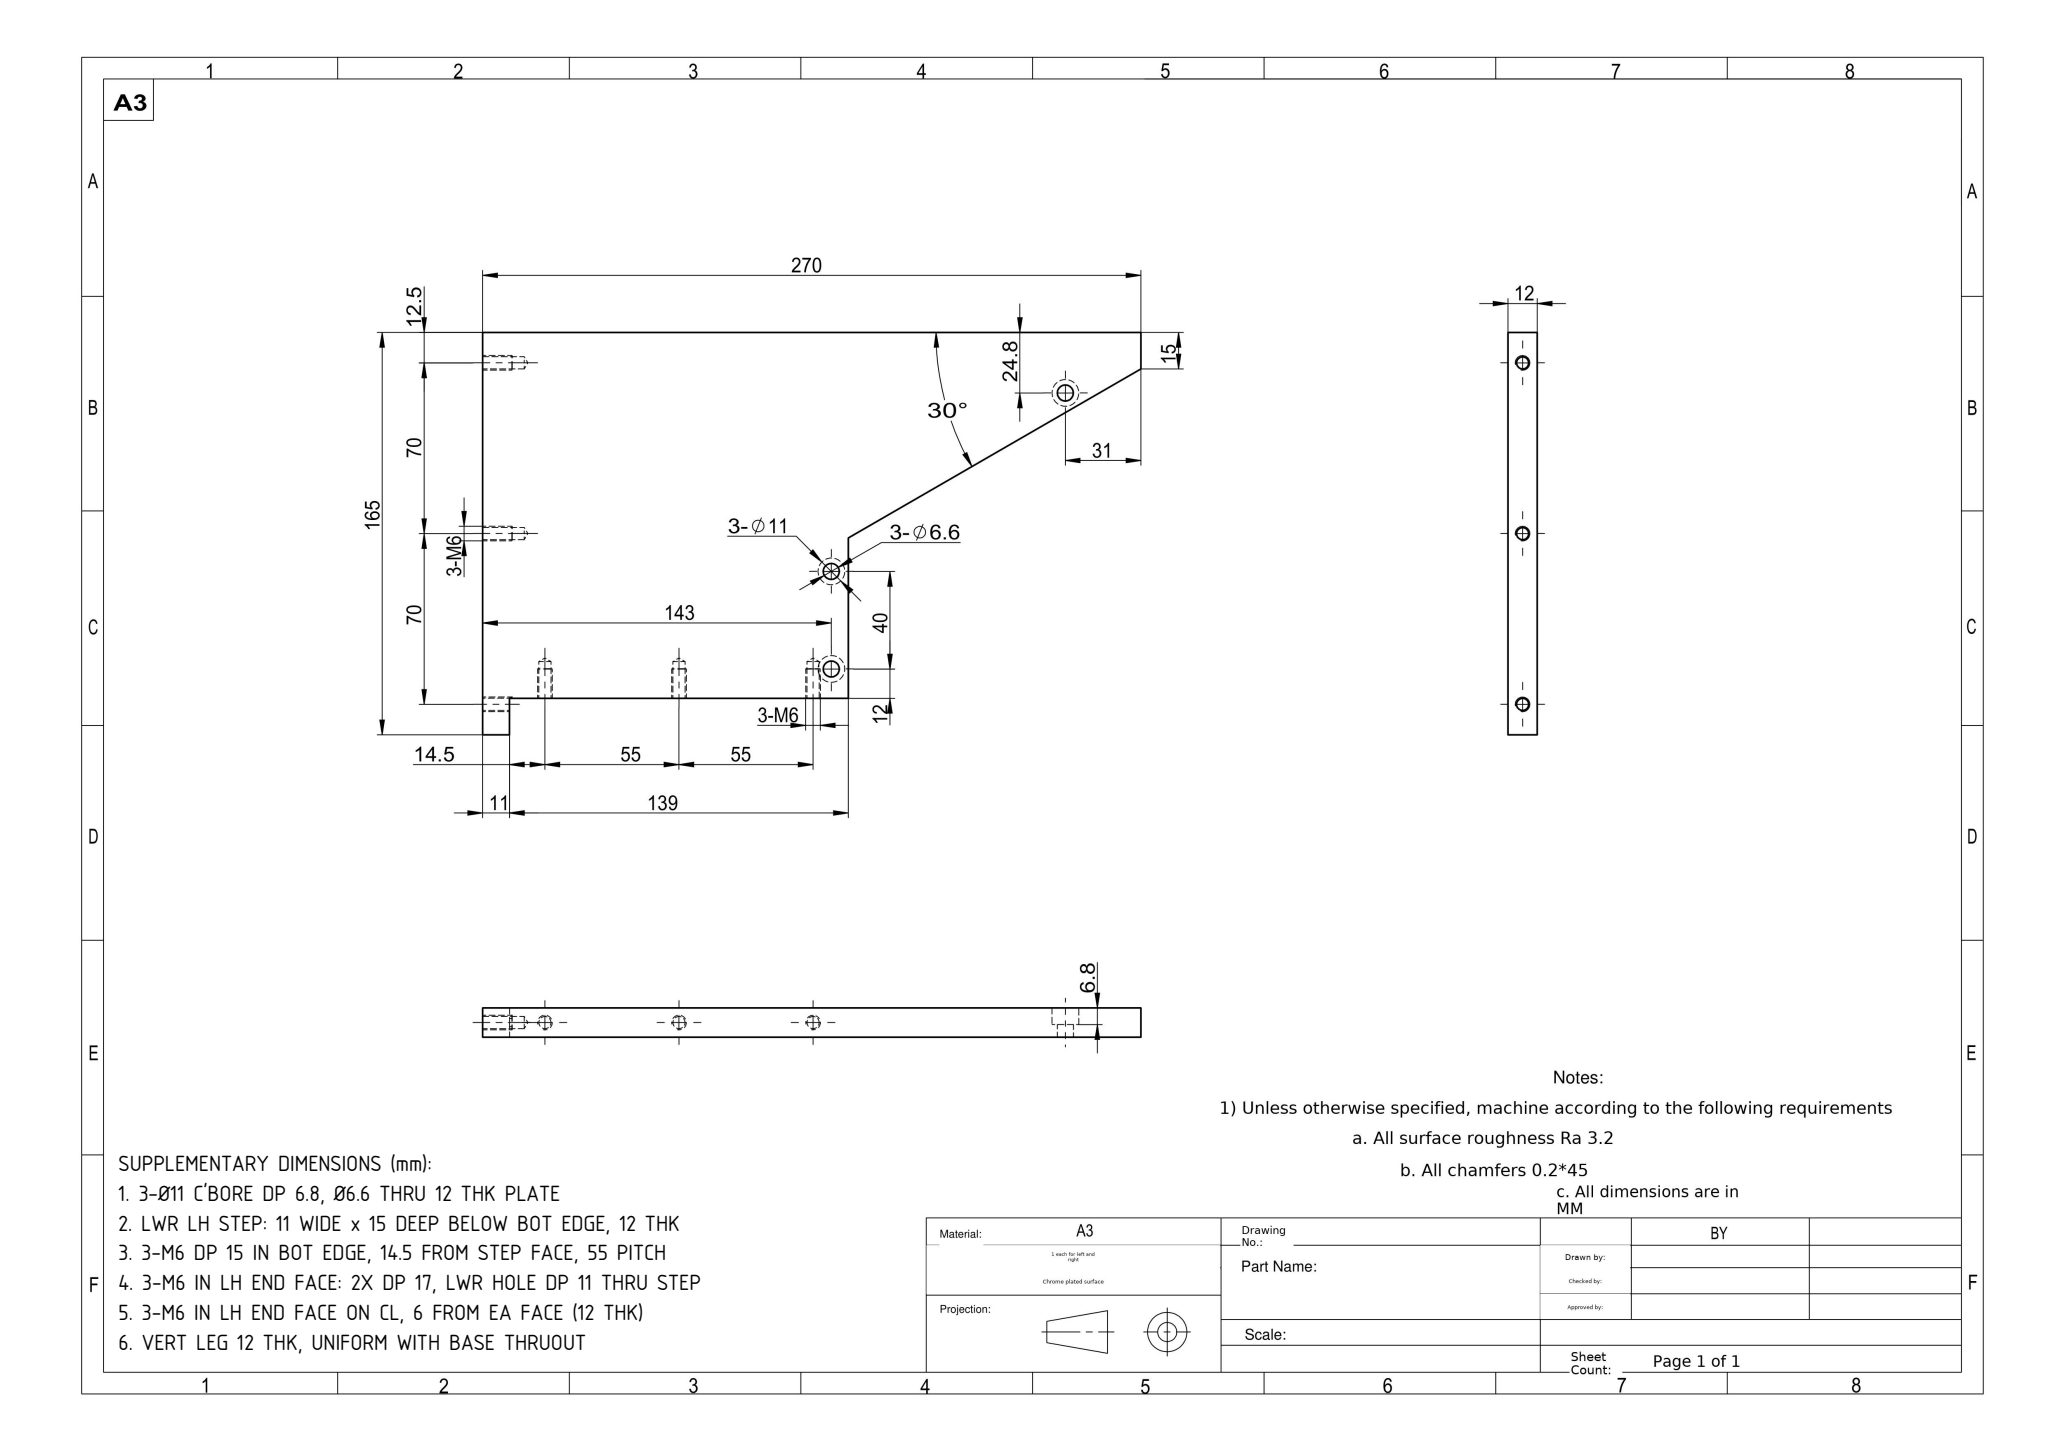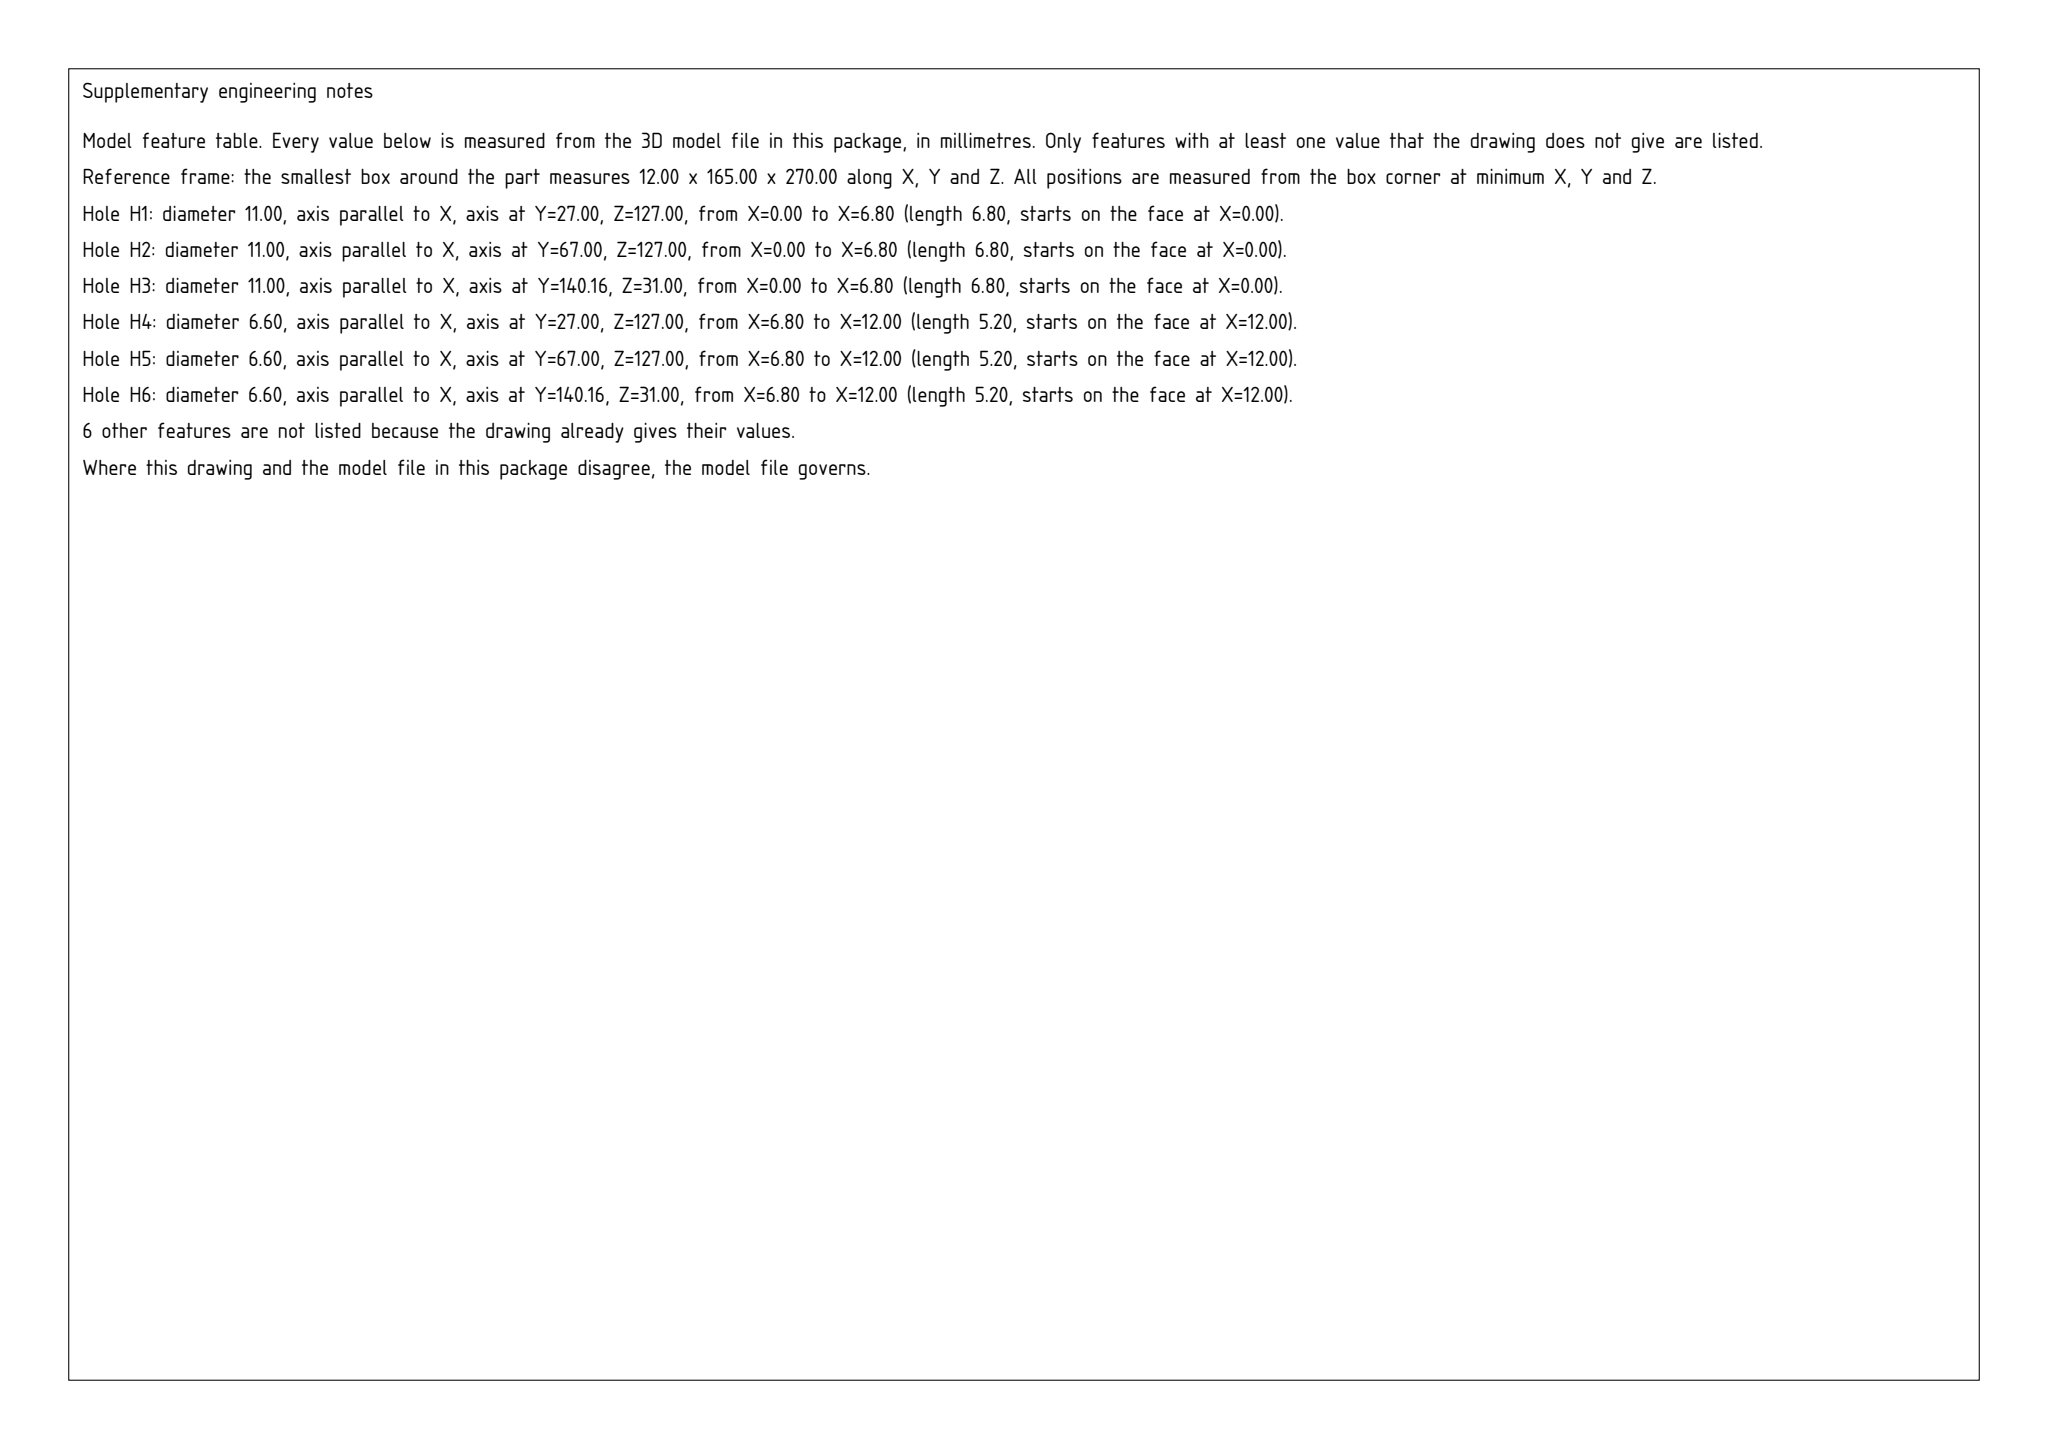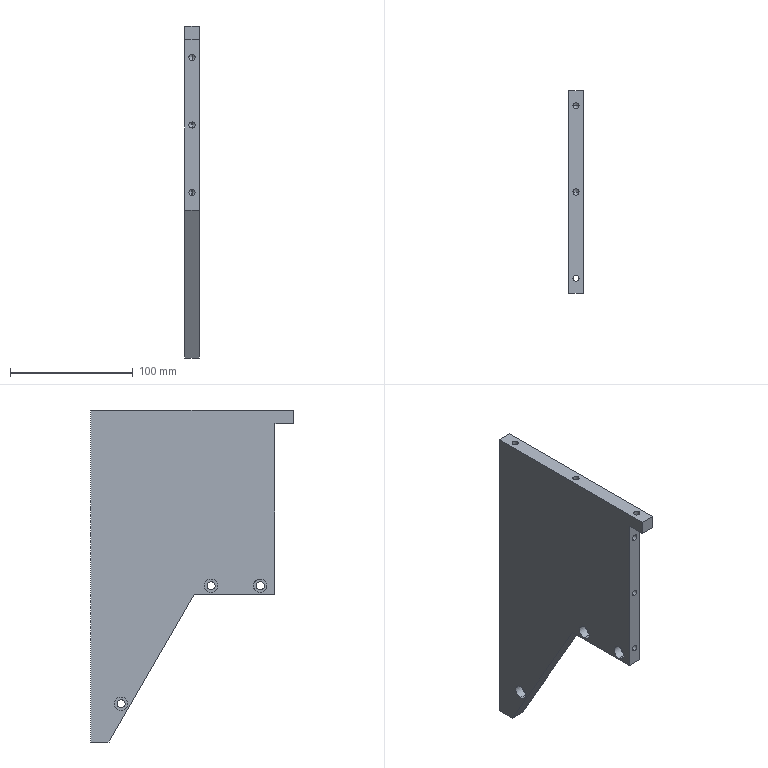Part | SolidWorks | mm | 1 solid | 47 faces | box 12 x 165 x 270 mm | volume 339177 mm3 | cylinder 24 | plane 13 | cone 10 | commonest cylinder face diameters 5 x12 6.6 x6 11 x6
build123d program:
from build123d import *

# Parameters (mm, degrees)
BOSS_EXTRUDE1_DEPTH                               = 6
SKETCH2_W                                         = 12
SKETCH2_H                                         = 11
BOSS_EXTRUDE2_DEPTH                               = 15
M6_TAPPED_HOLE1_D                                 = 5
M6_TAPPED_HOLE1_DEPTH                             = 17
M6_TAPPED_HOLE1_TIP                               = 1.502
M6_TAPPED_HOLE2_D                                 = 5
M6_TAPPED_HOLE2_DEPTH                             = 15
M6_TAPPED_HOLE2_TIP                               = 1.502
HOLE_SIZE_ACCORDING_TO_HEXAGON_SOCKET_D           = 6.6
HOLE_SIZE_ACCORDING_TO_HEXAGON_SOCKET_DEPTH       = 17
HOLE_SIZE_ACCORDING_TO_HEXAGON_SOCKET_CBORE_D     = 11
HOLE_SIZE_ACCORDING_TO_HEXAGON_SOCKET_CBORE_DEPTH = 6.8
HOLE_SIZE_ACCORDING_TO_HEXAGON_SOCKET_TIP         = 1.983


with BuildPart() as part:
    # Sketch1 → Boss-Extrude1 (new, symmetric)
    with BuildSketch(Plane(origin=(0, 0, 0), x_dir=(0, 0, -1), z_dir=(1, 0, 0))):
        Polygon((-75, 0), (75, 0), (75, 65.718), (195, 135), (195, 150), (-75, 150), align=None)
    extrude(amount=BOSS_EXTRUDE1_DEPTH, both=True)

    # Sketch2 → Boss-Extrude2 (add)
    with BuildSketch(Plane.XZ):
        with Locations((0, 69.5)):
            Rectangle(SKETCH2_W, SKETCH2_H)
    extrude(amount=BOSS_EXTRUDE2_DEPTH)

    # M6 Tapped Hole1
    with Locations(Plane.XY.offset(75)):
        with Locations((0, 137.5), (0, 67.5), (0, -2.5)):
            Hole(M6_TAPPED_HOLE1_D / 2, depth=M6_TAPPED_HOLE1_DEPTH)
            with Locations((0, 0, -(M6_TAPPED_HOLE1_DEPTH + M6_TAPPED_HOLE1_TIP / 2))):  # 118° drill point
                Cone(0, M6_TAPPED_HOLE1_D / 2, M6_TAPPED_HOLE1_TIP, mode=Mode.SUBTRACT)

    # M6 Tapped Hole2
    with Locations(Plane(origin=(0, 0, 0), x_dir=(-1, 0, 0), z_dir=(0, -1, 0))):
        with Locations((0, -49.5), (0, 5.5), (0, 60.5)):
            Hole(M6_TAPPED_HOLE2_D / 2, depth=M6_TAPPED_HOLE2_DEPTH)
            with Locations((0, 0, -(M6_TAPPED_HOLE2_DEPTH + M6_TAPPED_HOLE2_TIP / 2))):  # 118° drill point
                Cone(0, M6_TAPPED_HOLE2_D / 2, M6_TAPPED_HOLE2_TIP, mode=Mode.SUBTRACT)

    # Hole Size _ according to_ Hexagon Socket
    with Locations(Plane.ZY.offset(6)):
        with Locations((-68, 12), (-68, 52), (-163.996, 125.156)):
            CounterBoreHole(HOLE_SIZE_ACCORDING_TO_HEXAGON_SOCKET_D / 2, HOLE_SIZE_ACCORDING_TO_HEXAGON_SOCKET_CBORE_D / 2, HOLE_SIZE_ACCORDING_TO_HEXAGON_SOCKET_CBORE_DEPTH, depth=HOLE_SIZE_ACCORDING_TO_HEXAGON_SOCKET_DEPTH)
            with Locations((0, 0, -(HOLE_SIZE_ACCORDING_TO_HEXAGON_SOCKET_DEPTH + HOLE_SIZE_ACCORDING_TO_HEXAGON_SOCKET_TIP / 2))):  # 118° drill point
                Cone(0, HOLE_SIZE_ACCORDING_TO_HEXAGON_SOCKET_D / 2, HOLE_SIZE_ACCORDING_TO_HEXAGON_SOCKET_TIP, mode=Mode.SUBTRACT)


solid = part.part